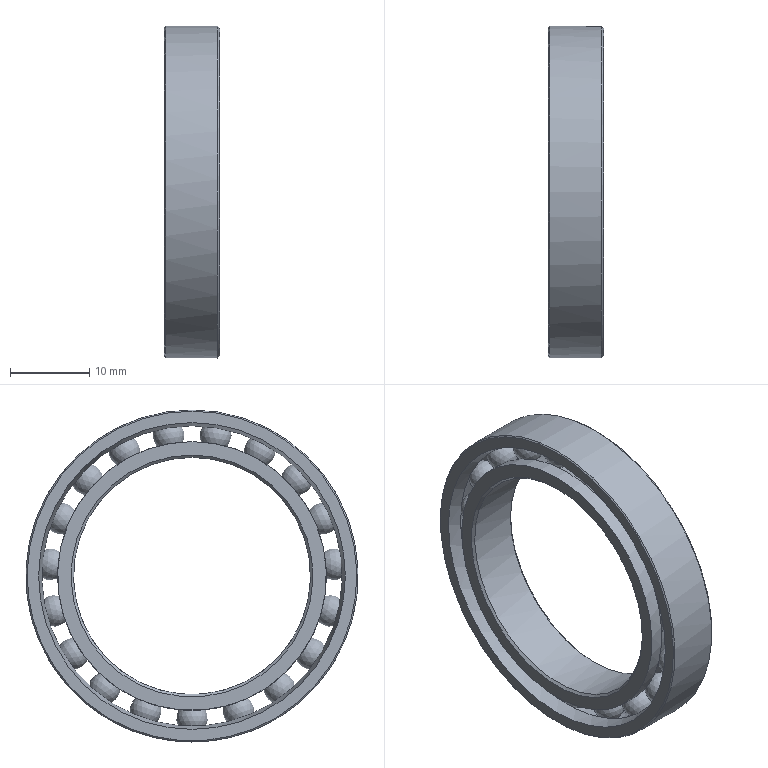Component | NX | GB-T292_C-1994_71806_C | 21 solids | 35 faces | volume 3189 mm3 | sphere 19 | cylinder 5 | cone 5 | plane 4 | torus 2 | commonest cylinder face diameters 34 x2 42 x1 38 x1 30 x1